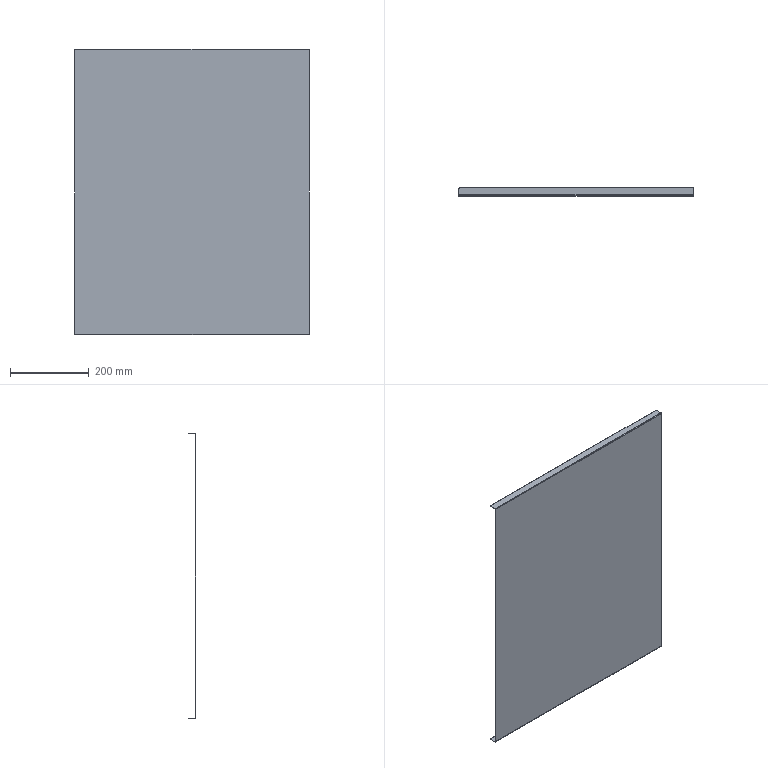Component | SolidWorks | DoorPlate-1_InnerDoorPanel-1 | 1 solid | 26 faces | volume 364310 mm3 | plane 22 | cylinder 4 | commonest cylinder face diameters 3.6 x2 2 x2 | material 304